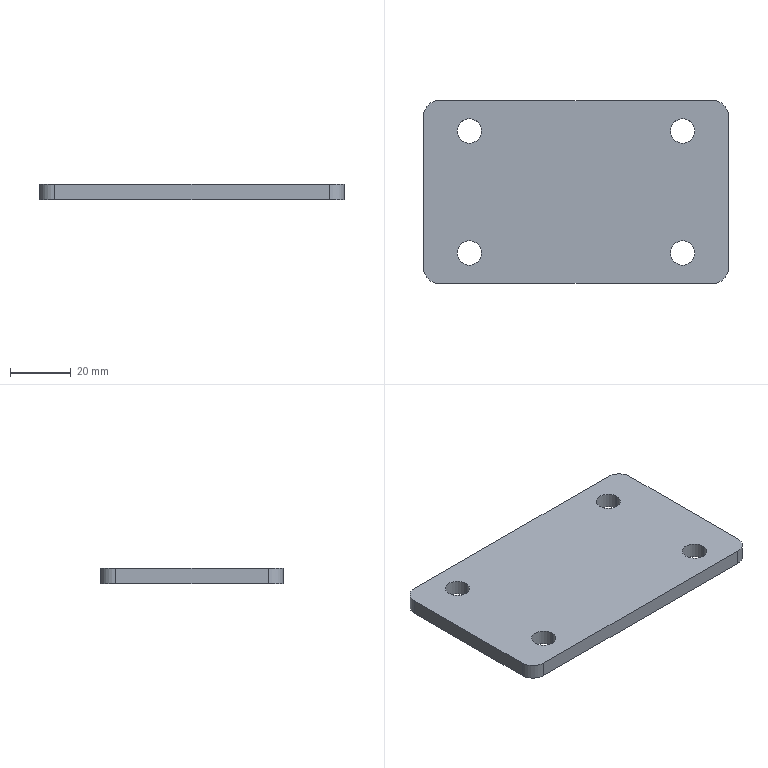Component | SolidWorks | VerticalMovingRectangularTubeWeldment-1_RectangularTubeWeldPlate3-2 | 1 solid | 18 faces | box 100 x 60 x 5 mm | volume 28887 mm3 | cylinder 12 | plane 6 | commonest cylinder face diameters 8 x8 10 x4 | material Plain Carbon Steel
STEP:
#1=COLOUR_RGB('',0.7922,0.8196,0.9333);
#2=FILL_AREA_STYLE_COLOUR('',#1);
#3=FILL_AREA_STYLE('',(#2));
#4=SURFACE_STYLE_FILL_AREA(#3);
#5=SURFACE_SIDE_STYLE('',(#4));
#6=SURFACE_STYLE_USAGE(.BOTH.,#5);
#7=PRESENTATION_STYLE_ASSIGNMENT((#6));
#8=CARTESIAN_POINT('',(-16.102,0.7874,12.205));
#9=VERTEX_POINT('',#8);
#10=CARTESIAN_POINT('',(-15.787,0.7874,12.205));
#11=VERTEX_POINT('',#10);
#12=CARTESIAN_POINT('',(-15.945,0.7874,12.205));
#13=DIRECTION('',(0.,0.,1.));
#14=DIRECTION('',(0.,-1.,0.));
#15=AXIS2_PLACEMENT_3D('',#12,#13,#14);
#16=CIRCLE('',#15,0.1575);
#17=EDGE_CURVE('',#9,#11,#16,.T.);
#18=ORIENTED_EDGE('',*,*,#17,.T.);
#19=CARTESIAN_POINT('',(-15.787,0.7874,12.008));
#20=VERTEX_POINT('',#19);
#21=CARTESIAN_POINT('',(-15.787,0.7874,12.008));
#22=DIRECTION('',(0.,0.,-1.));
#23=VECTOR('',#22,39.37);
#24=LINE('',#21,#23);
#25=EDGE_CURVE('',#11,#20,#24,.T.);
#26=ORIENTED_EDGE('',*,*,#25,.T.);
#27=CARTESIAN_POINT('',(-16.102,0.7874,12.008));
#28=VERTEX_POINT('',#27);
#29=CARTESIAN_POINT('',(-15.945,0.7874,12.008));
#30=DIRECTION('',(0.,0.,-1.));
#31=DIRECTION('',(-1.,0.,0.));
#32=AXIS2_PLACEMENT_3D('',#29,#30,#31);
#33=CIRCLE('',#32,0.1575);
#34=EDGE_CURVE('',#20,#28,#33,.T.);
#35=ORIENTED_EDGE('',*,*,#34,.T.);
#36=CARTESIAN_POINT('',(-16.102,0.7874,12.008));
#37=DIRECTION('',(0.,0.,-1.));
#38=VECTOR('',#37,39.37);
#39=LINE('',#36,#38);
#40=EDGE_CURVE('',#9,#28,#39,.T.);
#41=ORIENTED_EDGE('',*,*,#40,.F.);
#42=EDGE_LOOP('',(#18,#26,#35,#41));
#43=FACE_OUTER_BOUND('',#42,.T.);
#44=CARTESIAN_POINT('',(-15.945,0.7874,12.008));
#45=DIRECTION('',(0.,0.,-1.));
#46=DIRECTION('',(-1.,0.,0.));
#47=AXIS2_PLACEMENT_3D('',#44,#45,#46);
#48=CYLINDRICAL_SURFACE('',#47,0.1575);
#49=ADVANCED_FACE('',(#43),#48,.F.);
#50=CARTESIAN_POINT('',(-18.858,0.7874,12.205));
#51=VERTEX_POINT('',#50);
#52=CARTESIAN_POINT('',(-18.543,0.7874,12.205));
#53=VERTEX_POINT('',#52);
#54=CARTESIAN_POINT('',(-18.701,0.7874,12.205));
#55=DIRECTION('',(0.,0.,1.));
#56=DIRECTION('',(0.,-1.,0.));
#57=AXIS2_PLACEMENT_3D('',#54,#55,#56);
#58=CIRCLE('',#57,0.1575);
#59=EDGE_CURVE('',#51,#53,#58,.T.);
#60=ORIENTED_EDGE('',*,*,#59,.T.);
#61=CARTESIAN_POINT('',(-18.543,0.7874,12.008));
#62=VERTEX_POINT('',#61);
#63=CARTESIAN_POINT('',(-18.543,0.7874,12.008));
#64=DIRECTION('',(0.,0.,-1.));
#65=VECTOR('',#64,39.37);
#66=LINE('',#63,#65);
#67=EDGE_CURVE('',#53,#62,#66,.T.);
#68=ORIENTED_EDGE('',*,*,#67,.T.);
#69=CARTESIAN_POINT('',(-18.858,0.7874,12.008));
#70=VERTEX_POINT('',#69);
#71=CARTESIAN_POINT('',(-18.701,0.7874,12.008));
#72=DIRECTION('',(0.,0.,-1.));
#73=DIRECTION('',(-1.,0.,0.));
#74=AXIS2_PLACEMENT_3D('',#71,#72,#73);
#75=CIRCLE('',#74,0.1575);
#76=EDGE_CURVE('',#62,#70,#75,.T.);
#77=ORIENTED_EDGE('',*,*,#76,.T.);
#78=CARTESIAN_POINT('',(-18.858,0.7874,12.008));
#79=DIRECTION('',(0.,0.,-1.));
#80=VECTOR('',#79,39.37);
#81=LINE('',#78,#80);
#82=EDGE_CURVE('',#51,#70,#81,.T.);
#83=ORIENTED_EDGE('',*,*,#82,.F.);
#84=EDGE_LOOP('',(#60,#68,#77,#83));
#85=FACE_OUTER_BOUND('',#84,.T.);
#86=CARTESIAN_POINT('',(-18.701,0.7874,12.008));
#87=DIRECTION('',(0.,0.,-1.));
#88=DIRECTION('',(-1.,0.,0.));
#89=AXIS2_PLACEMENT_3D('',#86,#87,#88);
#90=CYLINDRICAL_SURFACE('',#89,0.1575);
#91=ADVANCED_FACE('',(#85),#90,.F.);
#92=CARTESIAN_POINT('',(-16.102,-0.7874,12.205));
#93=VERTEX_POINT('',#92);
#94=CARTESIAN_POINT('',(-15.787,-0.7874,12.205));
#95=VERTEX_POINT('',#94);
#96=CARTESIAN_POINT('',(-15.945,-0.7874,12.205));
#97=DIRECTION('',(0.,0.,1.));
#98=DIRECTION('',(0.,-1.,0.));
#99=AXIS2_PLACEMENT_3D('',#96,#97,#98);
#100=CIRCLE('',#99,0.1575);
#101=EDGE_CURVE('',#93,#95,#100,.T.);
#102=ORIENTED_EDGE('',*,*,#101,.T.);
#103=CARTESIAN_POINT('',(-15.787,-0.7874,12.008));
#104=VERTEX_POINT('',#103);
#105=CARTESIAN_POINT('',(-15.787,-0.7874,12.008));
#106=DIRECTION('',(0.,0.,-1.));
#107=VECTOR('',#106,39.37);
#108=LINE('',#105,#107);
#109=EDGE_CURVE('',#95,#104,#108,.T.);
#110=ORIENTED_EDGE('',*,*,#109,.T.);
#111=CARTESIAN_POINT('',(-16.102,-0.7874,12.008));
#112=VERTEX_POINT('',#111);
#113=CARTESIAN_POINT('',(-15.945,-0.7874,12.008));
#114=DIRECTION('',(0.,0.,-1.));
#115=DIRECTION('',(-1.,0.,0.));
#116=AXIS2_PLACEMENT_3D('',#113,#114,#115);
#117=CIRCLE('',#116,0.1575);
#118=EDGE_CURVE('',#104,#112,#117,.T.);
#119=ORIENTED_EDGE('',*,*,#118,.T.);
#120=CARTESIAN_POINT('',(-16.102,-0.7874,12.008));
#121=DIRECTION('',(0.,0.,-1.));
#122=VECTOR('',#121,39.37);
#123=LINE('',#120,#122);
#124=EDGE_CURVE('',#93,#112,#123,.T.);
#125=ORIENTED_EDGE('',*,*,#124,.F.);
#126=EDGE_LOOP('',(#102,#110,#119,#125));
#127=FACE_OUTER_BOUND('',#126,.T.);
#128=CARTESIAN_POINT('',(-15.945,-0.7874,12.008));
#129=DIRECTION('',(0.,0.,-1.));
#130=DIRECTION('',(-1.,0.,0.));
#131=AXIS2_PLACEMENT_3D('',#128,#129,#130);
#132=CYLINDRICAL_SURFACE('',#131,0.1575);
#133=ADVANCED_FACE('',(#127),#132,.F.);
#134=CARTESIAN_POINT('',(-18.858,-0.7874,12.205));
#135=VERTEX_POINT('',#134);
#136=CARTESIAN_POINT('',(-18.543,-0.7874,12.205));
#137=VERTEX_POINT('',#136);
#138=CARTESIAN_POINT('',(-18.701,-0.7874,12.205));
#139=DIRECTION('',(0.,0.,1.));
#140=DIRECTION('',(0.,-1.,0.));
#141=AXIS2_PLACEMENT_3D('',#138,#139,#140);
#142=CIRCLE('',#141,0.1575);
#143=EDGE_CURVE('',#135,#137,#142,.T.);
#144=ORIENTED_EDGE('',*,*,#143,.T.);
#145=CARTESIAN_POINT('',(-18.543,-0.7874,12.008));
#146=VERTEX_POINT('',#145);
#147=CARTESIAN_POINT('',(-18.543,-0.7874,12.008));
#148=DIRECTION('',(0.,0.,-1.));
#149=VECTOR('',#148,39.37);
#150=LINE('',#147,#149);
#151=EDGE_CURVE('',#137,#146,#150,.T.);
#152=ORIENTED_EDGE('',*,*,#151,.T.);
#153=CARTESIAN_POINT('',(-18.858,-0.7874,12.008));
#154=VERTEX_POINT('',#153);
#155=CARTESIAN_POINT('',(-18.701,-0.7874,12.008));
#156=DIRECTION('',(0.,0.,-1.));
#157=DIRECTION('',(-1.,0.,0.));
#158=AXIS2_PLACEMENT_3D('',#155,#156,#157);
#159=CIRCLE('',#158,0.1575);
#160=EDGE_CURVE('',#146,#154,#159,.T.);
#161=ORIENTED_EDGE('',*,*,#160,.T.);
#162=CARTESIAN_POINT('',(-18.858,-0.7874,12.008));
#163=DIRECTION('',(0.,0.,-1.));
#164=VECTOR('',#163,39.37);
#165=LINE('',#162,#164);
#166=EDGE_CURVE('',#135,#154,#165,.T.);
#167=ORIENTED_EDGE('',*,*,#166,.F.);
#168=EDGE_LOOP('',(#144,#152,#161,#167));
#169=FACE_OUTER_BOUND('',#168,.T.);
#170=CARTESIAN_POINT('',(-18.701,-0.7874,12.008));
#171=DIRECTION('',(0.,0.,-1.));
#172=DIRECTION('',(-1.,0.,0.));
#173=AXIS2_PLACEMENT_3D('',#170,#171,#172);
#174=CYLINDRICAL_SURFACE('',#173,0.1575);
#175=ADVANCED_FACE('',(#169),#174,.F.);
#176=CARTESIAN_POINT('',(-15.354,-0.9843,12.205));
#177=VERTEX_POINT('',#176);
#178=CARTESIAN_POINT('',(-15.354,0.9843,12.205));
#179=VERTEX_POINT('',#178);
#180=CARTESIAN_POINT('',(-15.354,1.181,12.205));
#181=DIRECTION('',(-0.,1.,0.));
#182=VECTOR('',#181,39.37);
#183=LINE('',#180,#182);
#184=EDGE_CURVE('',#177,#179,#183,.T.);
#185=ORIENTED_EDGE('',*,*,#184,.F.);
#186=CARTESIAN_POINT('',(-15.354,-0.9843,12.008));
#187=VERTEX_POINT('',#186);
#188=CARTESIAN_POINT('',(-15.354,-0.9843,12.205));
#189=DIRECTION('',(0.,0.,-1.));
#190=VECTOR('',#189,39.37);
#191=LINE('',#188,#190);
#192=EDGE_CURVE('',#177,#187,#191,.T.);
#193=ORIENTED_EDGE('',*,*,#192,.T.);
#194=CARTESIAN_POINT('',(-15.354,0.9843,12.008));
#195=VERTEX_POINT('',#194);
#196=CARTESIAN_POINT('',(-15.354,1.181,12.008));
#197=DIRECTION('',(-0.,1.,0.));
#198=VECTOR('',#197,39.37);
#199=LINE('',#196,#198);
#200=EDGE_CURVE('',#187,#195,#199,.T.);
#201=ORIENTED_EDGE('',*,*,#200,.T.);
#202=CARTESIAN_POINT('',(-15.354,0.9843,12.205));
#203=DIRECTION('',(0.,0.,1.));
#204=VECTOR('',#203,39.37);
#205=LINE('',#202,#204);
#206=EDGE_CURVE('',#195,#179,#205,.T.);
#207=ORIENTED_EDGE('',*,*,#206,.T.);
#208=EDGE_LOOP('',(#185,#193,#201,#207));
#209=FACE_OUTER_BOUND('',#208,.T.);
#210=CARTESIAN_POINT('',(-15.354,1.181,12.205));
#211=DIRECTION('',(-1.,-0.,0.));
#212=DIRECTION('',(0.,-1.,0.));
#213=AXIS2_PLACEMENT_3D('',#210,#211,#212);
#214=PLANE('',#213);
#215=ADVANCED_FACE('',(#209),#214,.F.);
#216=CARTESIAN_POINT('',(-15.551,1.181,12.008));
#217=VERTEX_POINT('',#216);
#218=CARTESIAN_POINT('',(-19.094,1.181,12.008));
#219=VERTEX_POINT('',#218);
#220=CARTESIAN_POINT('',(-19.291,1.181,12.008));
#221=DIRECTION('',(-1.,0.,0.));
#222=VECTOR('',#221,39.37);
#223=LINE('',#220,#222);
#224=EDGE_CURVE('',#217,#219,#223,.T.);
#225=ORIENTED_EDGE('',*,*,#224,.T.);
#226=CARTESIAN_POINT('',(-19.094,1.181,12.205));
#227=VERTEX_POINT('',#226);
#228=CARTESIAN_POINT('',(-19.094,1.181,12.205));
#229=DIRECTION('',(0.,0.,1.));
#230=VECTOR('',#229,39.37);
#231=LINE('',#228,#230);
#232=EDGE_CURVE('',#219,#227,#231,.T.);
#233=ORIENTED_EDGE('',*,*,#232,.T.);
#234=CARTESIAN_POINT('',(-15.551,1.181,12.205));
#235=VERTEX_POINT('',#234);
#236=CARTESIAN_POINT('',(-19.291,1.181,12.205));
#237=DIRECTION('',(-1.,0.,0.));
#238=VECTOR('',#237,39.37);
#239=LINE('',#236,#238);
#240=EDGE_CURVE('',#235,#227,#239,.T.);
#241=ORIENTED_EDGE('',*,*,#240,.F.);
#242=CARTESIAN_POINT('',(-15.551,1.181,12.205));
#243=DIRECTION('',(0.,0.,-1.));
#244=VECTOR('',#243,39.37);
#245=LINE('',#242,#244);
#246=EDGE_CURVE('',#235,#217,#245,.T.);
#247=ORIENTED_EDGE('',*,*,#246,.T.);
#248=EDGE_LOOP('',(#225,#233,#241,#247));
#249=FACE_OUTER_BOUND('',#248,.T.);
#250=CARTESIAN_POINT('',(-19.291,1.181,12.205));
#251=DIRECTION('',(0.,-1.,0.));
#252=DIRECTION('',(1.,0.,0.));
#253=AXIS2_PLACEMENT_3D('',#250,#251,#252);
#254=PLANE('',#253);
#255=ADVANCED_FACE('',(#249),#254,.F.);
#256=CARTESIAN_POINT('',(-19.291,0.9843,12.008));
#257=VERTEX_POINT('',#256);
#258=CARTESIAN_POINT('',(-19.291,-0.9843,12.008));
#259=VERTEX_POINT('',#258);
#260=CARTESIAN_POINT('',(-19.291,1.181,12.008));
#261=DIRECTION('',(0.,-1.,0.));
#262=VECTOR('',#261,39.37);
#263=LINE('',#260,#262);
#264=EDGE_CURVE('',#257,#259,#263,.T.);
#265=ORIENTED_EDGE('',*,*,#264,.T.);
#266=CARTESIAN_POINT('',(-19.291,-0.9843,12.205));
#267=VERTEX_POINT('',#266);
#268=CARTESIAN_POINT('',(-19.291,-0.9843,12.205));
#269=DIRECTION('',(0.,0.,1.));
#270=VECTOR('',#269,39.37);
#271=LINE('',#268,#270);
#272=EDGE_CURVE('',#259,#267,#271,.T.);
#273=ORIENTED_EDGE('',*,*,#272,.T.);
#274=CARTESIAN_POINT('',(-19.291,0.9843,12.205));
#275=VERTEX_POINT('',#274);
#276=CARTESIAN_POINT('',(-19.291,1.181,12.205));
#277=DIRECTION('',(0.,-1.,0.));
#278=VECTOR('',#277,39.37);
#279=LINE('',#276,#278);
#280=EDGE_CURVE('',#275,#267,#279,.T.);
#281=ORIENTED_EDGE('',*,*,#280,.F.);
#282=CARTESIAN_POINT('',(-19.291,0.9843,12.205));
#283=DIRECTION('',(0.,0.,-1.));
#284=VECTOR('',#283,39.37);
#285=LINE('',#282,#284);
#286=EDGE_CURVE('',#275,#257,#285,.T.);
#287=ORIENTED_EDGE('',*,*,#286,.T.);
#288=EDGE_LOOP('',(#265,#273,#281,#287));
#289=FACE_OUTER_BOUND('',#288,.T.);
#290=CARTESIAN_POINT('',(-19.291,1.181,12.205));
#291=DIRECTION('',(1.,0.,0.));
#292=DIRECTION('',(-0.,1.,0.));
#293=AXIS2_PLACEMENT_3D('',#290,#291,#292);
#294=PLANE('',#293);
#295=ADVANCED_FACE('',(#289),#294,.F.);
#296=CARTESIAN_POINT('',(-19.094,-1.181,12.008));
#297=VERTEX_POINT('',#296);
#298=CARTESIAN_POINT('',(-15.551,-1.181,12.008));
#299=VERTEX_POINT('',#298);
#300=CARTESIAN_POINT('',(-19.291,-1.181,12.008));
#301=DIRECTION('',(1.,0.,0.));
#302=VECTOR('',#301,39.37);
#303=LINE('',#300,#302);
#304=EDGE_CURVE('',#297,#299,#303,.T.);
#305=ORIENTED_EDGE('',*,*,#304,.T.);
#306=CARTESIAN_POINT('',(-15.551,-1.181,12.205));
#307=VERTEX_POINT('',#306);
#308=CARTESIAN_POINT('',(-15.551,-1.181,12.205));
#309=DIRECTION('',(0.,0.,1.));
#310=VECTOR('',#309,39.37);
#311=LINE('',#308,#310);
#312=EDGE_CURVE('',#299,#307,#311,.T.);
#313=ORIENTED_EDGE('',*,*,#312,.T.);
#314=CARTESIAN_POINT('',(-19.094,-1.181,12.205));
#315=VERTEX_POINT('',#314);
#316=CARTESIAN_POINT('',(-19.291,-1.181,12.205));
#317=DIRECTION('',(1.,0.,0.));
#318=VECTOR('',#317,39.37);
#319=LINE('',#316,#318);
#320=EDGE_CURVE('',#315,#307,#319,.T.);
#321=ORIENTED_EDGE('',*,*,#320,.F.);
#322=CARTESIAN_POINT('',(-19.094,-1.181,12.205));
#323=DIRECTION('',(0.,0.,-1.));
#324=VECTOR('',#323,39.37);
#325=LINE('',#322,#324);
#326=EDGE_CURVE('',#315,#297,#325,.T.);
#327=ORIENTED_EDGE('',*,*,#326,.T.);
#328=EDGE_LOOP('',(#305,#313,#321,#327));
#329=FACE_OUTER_BOUND('',#328,.T.);
#330=CARTESIAN_POINT('',(-19.291,-1.181,12.205));
#331=DIRECTION('',(0.,1.,0.));
#332=DIRECTION('',(-1.,0.,0.));
#333=AXIS2_PLACEMENT_3D('',#330,#331,#332);
#334=PLANE('',#333);
#335=ADVANCED_FACE('',(#329),#334,.F.);
#336=ORIENTED_EDGE('',*,*,#17,.F.);
#337=CARTESIAN_POINT('',(-15.945,0.7874,12.205));
#338=DIRECTION('',(0.,0.,1.));
#339=DIRECTION('',(0.,-1.,0.));
#340=AXIS2_PLACEMENT_3D('',#337,#338,#339);
#341=CIRCLE('',#340,0.1575);
#342=EDGE_CURVE('',#11,#9,#341,.T.);
#343=ORIENTED_EDGE('',*,*,#342,.F.);
#344=EDGE_LOOP('',(#336,#343));
#345=FACE_BOUND('',#344,.T.);
#346=ORIENTED_EDGE('',*,*,#59,.F.);
#347=CARTESIAN_POINT('',(-18.701,0.7874,12.205));
#348=DIRECTION('',(0.,0.,1.));
#349=DIRECTION('',(0.,-1.,0.));
#350=AXIS2_PLACEMENT_3D('',#347,#348,#349);
#351=CIRCLE('',#350,0.1575);
#352=EDGE_CURVE('',#53,#51,#351,.T.);
#353=ORIENTED_EDGE('',*,*,#352,.F.);
#354=EDGE_LOOP('',(#346,#353));
#355=FACE_BOUND('',#354,.T.);
#356=ORIENTED_EDGE('',*,*,#101,.F.);
#357=CARTESIAN_POINT('',(-15.945,-0.7874,12.205));
#358=DIRECTION('',(0.,0.,1.));
#359=DIRECTION('',(0.,-1.,0.));
#360=AXIS2_PLACEMENT_3D('',#357,#358,#359);
#361=CIRCLE('',#360,0.1575);
#362=EDGE_CURVE('',#95,#93,#361,.T.);
#363=ORIENTED_EDGE('',*,*,#362,.F.);
#364=EDGE_LOOP('',(#356,#363));
#365=FACE_BOUND('',#364,.T.);
#366=ORIENTED_EDGE('',*,*,#143,.F.);
#367=CARTESIAN_POINT('',(-18.701,-0.7874,12.205));
#368=DIRECTION('',(0.,0.,1.));
#369=DIRECTION('',(0.,-1.,0.));
#370=AXIS2_PLACEMENT_3D('',#367,#368,#369);
#371=CIRCLE('',#370,0.1575);
#372=EDGE_CURVE('',#137,#135,#371,.T.);
#373=ORIENTED_EDGE('',*,*,#372,.F.);
#374=EDGE_LOOP('',(#366,#373));
#375=FACE_BOUND('',#374,.T.);
#376=ORIENTED_EDGE('',*,*,#320,.T.);
#377=CARTESIAN_POINT('',(-15.551,-0.9843,12.205));
#378=DIRECTION('',(0.,0.,1.));
#379=DIRECTION('',(0.,-1.,0.));
#380=AXIS2_PLACEMENT_3D('',#377,#378,#379);
#381=CIRCLE('',#380,0.1969);
#382=EDGE_CURVE('',#307,#177,#381,.T.);
#383=ORIENTED_EDGE('',*,*,#382,.T.);
#384=ORIENTED_EDGE('',*,*,#184,.T.);
#385=CARTESIAN_POINT('',(-15.551,0.9843,12.205));
#386=DIRECTION('',(0.,0.,1.));
#387=DIRECTION('',(0.,-1.,0.));
#388=AXIS2_PLACEMENT_3D('',#385,#386,#387);
#389=CIRCLE('',#388,0.1969);
#390=EDGE_CURVE('',#179,#235,#389,.T.);
#391=ORIENTED_EDGE('',*,*,#390,.T.);
#392=ORIENTED_EDGE('',*,*,#240,.T.);
#393=CARTESIAN_POINT('',(-19.094,0.9843,12.205));
#394=DIRECTION('',(0.,0.,1.));
#395=DIRECTION('',(0.,-1.,0.));
#396=AXIS2_PLACEMENT_3D('',#393,#394,#395);
#397=CIRCLE('',#396,0.1969);
#398=EDGE_CURVE('',#227,#275,#397,.T.);
#399=ORIENTED_EDGE('',*,*,#398,.T.);
#400=ORIENTED_EDGE('',*,*,#280,.T.);
#401=CARTESIAN_POINT('',(-19.094,-0.9843,12.205));
#402=DIRECTION('',(0.,0.,1.));
#403=DIRECTION('',(0.,-1.,0.));
#404=AXIS2_PLACEMENT_3D('',#401,#402,#403);
#405=CIRCLE('',#404,0.1969);
#406=EDGE_CURVE('',#267,#315,#405,.T.);
#407=ORIENTED_EDGE('',*,*,#406,.T.);
#408=EDGE_LOOP('',(#376,#383,#384,#391,#392,#399,#400,#407));
#409=FACE_OUTER_BOUND('',#408,.T.);
#410=CARTESIAN_POINT('',(-17.323,-0.,12.205));
#411=DIRECTION('',(0.,0.,1.));
#412=DIRECTION('',(0.,-1.,0.));
#413=AXIS2_PLACEMENT_3D('',#410,#411,#412);
#414=PLANE('',#413);
#415=ADVANCED_FACE('',(#345,#355,#365,#375,#409),#414,.T.);
#416=CARTESIAN_POINT('',(-15.945,0.7874,12.008));
#417=DIRECTION('',(0.,0.,-1.));
#418=DIRECTION('',(-1.,0.,0.));
#419=AXIS2_PLACEMENT_3D('',#416,#417,#418);
#420=CIRCLE('',#419,0.1575);
#421=EDGE_CURVE('',#28,#20,#420,.T.);
#422=ORIENTED_EDGE('',*,*,#421,.F.);
#423=ORIENTED_EDGE('',*,*,#34,.F.);
#424=EDGE_LOOP('',(#422,#423));
#425=FACE_BOUND('',#424,.T.);
#426=CARTESIAN_POINT('',(-18.701,0.7874,12.008));
#427=DIRECTION('',(0.,0.,-1.));
#428=DIRECTION('',(-1.,0.,0.));
#429=AXIS2_PLACEMENT_3D('',#426,#427,#428);
#430=CIRCLE('',#429,0.1575);
#431=EDGE_CURVE('',#70,#62,#430,.T.);
#432=ORIENTED_EDGE('',*,*,#431,.F.);
#433=ORIENTED_EDGE('',*,*,#76,.F.);
#434=EDGE_LOOP('',(#432,#433));
#435=FACE_BOUND('',#434,.T.);
#436=CARTESIAN_POINT('',(-15.945,-0.7874,12.008));
#437=DIRECTION('',(0.,0.,-1.));
#438=DIRECTION('',(-1.,0.,0.));
#439=AXIS2_PLACEMENT_3D('',#436,#437,#438);
#440=CIRCLE('',#439,0.1575);
#441=EDGE_CURVE('',#112,#104,#440,.T.);
#442=ORIENTED_EDGE('',*,*,#441,.F.);
#443=ORIENTED_EDGE('',*,*,#118,.F.);
#444=EDGE_LOOP('',(#442,#443));
#445=FACE_BOUND('',#444,.T.);
#446=CARTESIAN_POINT('',(-18.701,-0.7874,12.008));
#447=DIRECTION('',(0.,0.,-1.));
#448=DIRECTION('',(-1.,0.,0.));
#449=AXIS2_PLACEMENT_3D('',#446,#447,#448);
#450=CIRCLE('',#449,0.1575);
#451=EDGE_CURVE('',#154,#146,#450,.T.);
#452=ORIENTED_EDGE('',*,*,#451,.F.);
#453=ORIENTED_EDGE('',*,*,#160,.F.);
#454=EDGE_LOOP('',(#452,#453));
#455=FACE_BOUND('',#454,.T.);
#456=ORIENTED_EDGE('',*,*,#200,.F.);
#457=CARTESIAN_POINT('',(-15.551,-0.9843,12.008));
#458=DIRECTION('',(0.,0.,-1.));
#459=DIRECTION('',(0.,-1.,0.));
#460=AXIS2_PLACEMENT_3D('',#457,#458,#459);
#461=CIRCLE('',#460,0.1969);
#462=EDGE_CURVE('',#187,#299,#461,.T.);
#463=ORIENTED_EDGE('',*,*,#462,.T.);
#464=ORIENTED_EDGE('',*,*,#304,.F.);
#465=CARTESIAN_POINT('',(-19.094,-0.9843,12.008));
#466=DIRECTION('',(0.,0.,-1.));
#467=DIRECTION('',(0.,-1.,0.));
#468=AXIS2_PLACEMENT_3D('',#465,#466,#467);
#469=CIRCLE('',#468,0.1969);
#470=EDGE_CURVE('',#297,#259,#469,.T.);
#471=ORIENTED_EDGE('',*,*,#470,.T.);
#472=ORIENTED_EDGE('',*,*,#264,.F.);
#473=CARTESIAN_POINT('',(-19.094,0.9843,12.008));
#474=DIRECTION('',(0.,0.,-1.));
#475=DIRECTION('',(0.,-1.,0.));
#476=AXIS2_PLACEMENT_3D('',#473,#474,#475);
#477=CIRCLE('',#476,0.1969);
#478=EDGE_CURVE('',#257,#219,#477,.T.);
#479=ORIENTED_EDGE('',*,*,#478,.T.);
#480=ORIENTED_EDGE('',*,*,#224,.F.);
#481=CARTESIAN_POINT('',(-15.551,0.9843,12.008));
#482=DIRECTION('',(0.,0.,-1.));
#483=DIRECTION('',(0.,-1.,0.));
#484=AXIS2_PLACEMENT_3D('',#481,#482,#483);
#485=CIRCLE('',#484,0.1969);
#486=EDGE_CURVE('',#217,#195,#485,.T.);
#487=ORIENTED_EDGE('',*,*,#486,.T.);
#488=EDGE_LOOP('',(#456,#463,#464,#471,#472,#479,#480,#487));
#489=FACE_OUTER_BOUND('',#488,.T.);
#490=CARTESIAN_POINT('',(-17.323,-0.,12.008));
#491=DIRECTION('',(0.,0.,1.));
#492=DIRECTION('',(0.,-1.,0.));
#493=AXIS2_PLACEMENT_3D('',#490,#491,#492);
#494=PLANE('',#493);
#495=ADVANCED_FACE('',(#425,#435,#445,#455,#489),#494,.F.);
#496=ORIENTED_EDGE('',*,*,#382,.F.);
#497=ORIENTED_EDGE('',*,*,#312,.F.);
#498=ORIENTED_EDGE('',*,*,#462,.F.);
#499=ORIENTED_EDGE('',*,*,#192,.F.);
#500=EDGE_LOOP('',(#496,#497,#498,#499));
#501=FACE_OUTER_BOUND('',#500,.T.);
#502=CARTESIAN_POINT('',(-15.551,-0.9843,12.205));
#503=DIRECTION('',(0.,0.,-1.));
#504=DIRECTION('',(0.,1.,0.));
#505=AXIS2_PLACEMENT_3D('',#502,#503,#504);
#506=CYLINDRICAL_SURFACE('',#505,0.1969);
#507=ADVANCED_FACE('',(#501),#506,.T.);
#508=ORIENTED_EDGE('',*,*,#406,.F.);
#509=ORIENTED_EDGE('',*,*,#272,.F.);
#510=ORIENTED_EDGE('',*,*,#470,.F.);
#511=ORIENTED_EDGE('',*,*,#326,.F.);
#512=EDGE_LOOP('',(#508,#509,#510,#511));
#513=FACE_OUTER_BOUND('',#512,.T.);
#514=CARTESIAN_POINT('',(-19.094,-0.9843,12.205));
#515=DIRECTION('',(0.,0.,-1.));
#516=DIRECTION('',(0.,1.,0.));
#517=AXIS2_PLACEMENT_3D('',#514,#515,#516);
#518=CYLINDRICAL_SURFACE('',#517,0.1969);
#519=ADVANCED_FACE('',(#513),#518,.T.);
#520=ORIENTED_EDGE('',*,*,#398,.F.);
#521=ORIENTED_EDGE('',*,*,#232,.F.);
#522=ORIENTED_EDGE('',*,*,#478,.F.);
#523=ORIENTED_EDGE('',*,*,#286,.F.);
#524=EDGE_LOOP('',(#520,#521,#522,#523));
#525=FACE_OUTER_BOUND('',#524,.T.);
#526=CARTESIAN_POINT('',(-19.094,0.9843,12.205));
#527=DIRECTION('',(0.,0.,-1.));
#528=DIRECTION('',(0.,1.,0.));
#529=AXIS2_PLACEMENT_3D('',#526,#527,#528);
#530=CYLINDRICAL_SURFACE('',#529,0.1969);
#531=ADVANCED_FACE('',(#525),#530,.T.);
#532=ORIENTED_EDGE('',*,*,#390,.F.);
#533=ORIENTED_EDGE('',*,*,#206,.F.);
#534=ORIENTED_EDGE('',*,*,#486,.F.);
#535=ORIENTED_EDGE('',*,*,#246,.F.);
#536=EDGE_LOOP('',(#532,#533,#534,#535));
#537=FACE_OUTER_BOUND('',#536,.T.);
#538=CARTESIAN_POINT('',(-15.551,0.9843,12.205));
#539=DIRECTION('',(0.,0.,-1.));
#540=DIRECTION('',(0.,1.,0.));
#541=AXIS2_PLACEMENT_3D('',#538,#539,#540);
#542=CYLINDRICAL_SURFACE('',#541,0.1969);
#543=ADVANCED_FACE('',(#537),#542,.T.);
#544=ORIENTED_EDGE('',*,*,#151,.F.);
#545=ORIENTED_EDGE('',*,*,#372,.T.);
#546=ORIENTED_EDGE('',*,*,#166,.T.);
#547=ORIENTED_EDGE('',*,*,#451,.T.);
#548=EDGE_LOOP('',(#544,#545,#546,#547));
#549=FACE_OUTER_BOUND('',#548,.T.);
#550=CARTESIAN_POINT('',(-18.701,-0.7874,12.008));
#551=DIRECTION('',(0.,0.,-1.));
#552=DIRECTION('',(-1.,0.,0.));
#553=AXIS2_PLACEMENT_3D('',#550,#551,#552);
#554=CYLINDRICAL_SURFACE('',#553,0.1575);
#555=ADVANCED_FACE('',(#549),#554,.F.);
#556=ORIENTED_EDGE('',*,*,#109,.F.);
#557=ORIENTED_EDGE('',*,*,#362,.T.);
#558=ORIENTED_EDGE('',*,*,#124,.T.);
#559=ORIENTED_EDGE('',*,*,#441,.T.);
#560=EDGE_LOOP('',(#556,#557,#558,#559));
#561=FACE_OUTER_BOUND('',#560,.T.);
#562=CARTESIAN_POINT('',(-15.945,-0.7874,12.008));
#563=DIRECTION('',(0.,0.,-1.));
#564=DIRECTION('',(-1.,0.,0.));
#565=AXIS2_PLACEMENT_3D('',#562,#563,#564);
#566=CYLINDRICAL_SURFACE('',#565,0.1575);
#567=ADVANCED_FACE('',(#561),#566,.F.);
#568=ORIENTED_EDGE('',*,*,#67,.F.);
#569=ORIENTED_EDGE('',*,*,#352,.T.);
#570=ORIENTED_EDGE('',*,*,#82,.T.);
#571=ORIENTED_EDGE('',*,*,#431,.T.);
#572=EDGE_LOOP('',(#568,#569,#570,#571));
#573=FACE_OUTER_BOUND('',#572,.T.);
#574=CARTESIAN_POINT('',(-18.701,0.7874,12.008));
#575=DIRECTION('',(0.,0.,-1.));
#576=DIRECTION('',(-1.,0.,0.));
#577=AXIS2_PLACEMENT_3D('',#574,#575,#576);
#578=CYLINDRICAL_SURFACE('',#577,0.1575);
#579=ADVANCED_FACE('',(#573),#578,.F.);
#580=ORIENTED_EDGE('',*,*,#25,.F.);
#581=ORIENTED_EDGE('',*,*,#342,.T.);
#582=ORIENTED_EDGE('',*,*,#40,.T.);
#583=ORIENTED_EDGE('',*,*,#421,.T.);
#584=EDGE_LOOP('',(#580,#581,#582,#583));
#585=FACE_OUTER_BOUND('',#584,.T.);
#586=CARTESIAN_POINT('',(-15.945,0.7874,12.008));
#587=DIRECTION('',(0.,0.,-1.));
#588=DIRECTION('',(-1.,0.,0.));
#589=AXIS2_PLACEMENT_3D('',#586,#587,#588);
#590=CYLINDRICAL_SURFACE('',#589,0.1575);
#591=ADVANCED_FACE('',(#585),#590,.F.);
#592=CLOSED_SHELL('',(#49,#91,#133,#175,#215,#255,#295,#335,#415,#495,#507,#519,#531,#543,#555,#567,#579,#591));
#593=MANIFOLD_SOLID_BREP('',#592);
#594=STYLED_ITEM('',(#7),#593);
#595=(LENGTH_UNIT()NAMED_UNIT(*)SI_UNIT($,.METRE.));
#596=LENGTH_MEASURE_WITH_UNIT(LENGTH_MEASURE(0.0254),#595);
#597=DIMENSIONAL_EXPONENTS(1.,0.,0.,0.,0.,0.,0.);
#598=(CONVERSION_BASED_UNIT('',#596)LENGTH_UNIT()NAMED_UNIT(#597));
#599=UNCERTAINTY_MEASURE_WITH_UNIT(LENGTH_MEASURE(0.00001),#598,'','');
#600=(NAMED_UNIT(*)PLANE_ANGLE_UNIT()SI_UNIT($,.RADIAN.));
#601=(NAMED_UNIT(*)SI_UNIT($,.STERADIAN.)SOLID_ANGLE_UNIT());
#602=(GEOMETRIC_REPRESENTATION_CONTEXT(3)GLOBAL_UNCERTAINTY_ASSIGNED_CONTEXT((#599))GLOBAL_UNIT_ASSIGNED_CONTEXT((#598,#600,#601))REPRESENTATION_CONTEXT('',''));
#603=MECHANICAL_DESIGN_GEOMETRIC_PRESENTATION_REPRESENTATION('',(#594),#602);
#604=PRESENTATION_LAYER_ASSIGNMENT('','',(#594));
#605=CARTESIAN_POINT('',(0.,0.,0.));
#606=DIRECTION('',(0.,0.,1.));
#607=DIRECTION('',(1.,0.,0.));
#608=AXIS2_PLACEMENT_3D('',#605,#606,#607);
#609=(LENGTH_UNIT()NAMED_UNIT(*)SI_UNIT($,.METRE.));
#610=LENGTH_MEASURE_WITH_UNIT(LENGTH_MEASURE(0.0254),#609);
#611=DIMENSIONAL_EXPONENTS(1.,0.,0.,0.,0.,0.,0.);
#612=(CONVERSION_BASED_UNIT('',#610)LENGTH_UNIT()NAMED_UNIT(#611));
#613=UNCERTAINTY_MEASURE_WITH_UNIT(LENGTH_MEASURE(0.00001),#612,'','');
#614=(NAMED_UNIT(*)PLANE_ANGLE_UNIT()SI_UNIT($,.RADIAN.));
#615=(NAMED_UNIT(*)SI_UNIT($,.STERADIAN.)SOLID_ANGLE_UNIT());
#616=(GEOMETRIC_REPRESENTATION_CONTEXT(3)GLOBAL_UNCERTAINTY_ASSIGNED_CONTEXT((#613))GLOBAL_UNIT_ASSIGNED_CONTEXT((#612,#614,#615))REPRESENTATION_CONTEXT('',''));
#617=ADVANCED_BREP_SHAPE_REPRESENTATION('',(#593,#608),#616);